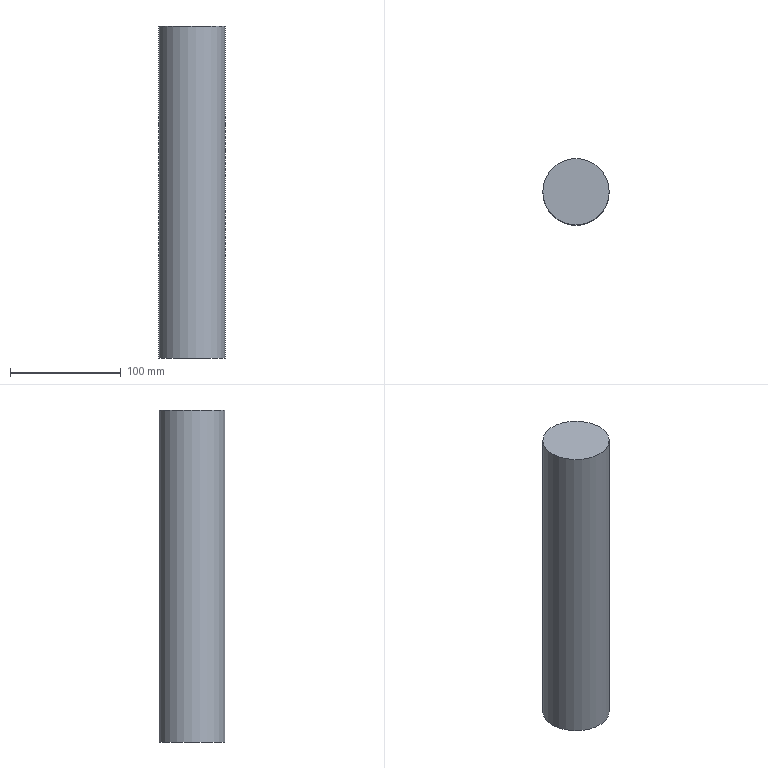Component | NX | CONNECTING_ROD | 1 solid | 3 faces | box 60 x 60 x 300 mm | volume 848230 mm3 | plane 2 | cylinder 1 | commonest cylinder face diameters 60 x1
STEP:
#1=CARTESIAN_POINT('',(0.,0.,0.));
#2=DIRECTION('',(0.,0.,1.));
#3=DIRECTION('',(1.,0.,0.));
#4=AXIS2_PLACEMENT_3D('',#1,#2,#3);
#5=CARTESIAN_POINT('',(30.,0.,-672.5));
#6=VERTEX_POINT('',#5);
#7=CARTESIAN_POINT('',(0.,0.,-672.5));
#8=DIRECTION('',(0.,0.,1.));
#9=DIRECTION('',(1.,0.,0.));
#10=AXIS2_PLACEMENT_3D('',#7,#8,#9);
#11=CIRCLE('',#10,30.);
#12=CARTESIAN_POINT('',(0.,0.,-672.5));
#13=DIRECTION('',(0.,0.,-1.));
#14=DIRECTION('',(1.,0.,0.));
#15=AXIS2_PLACEMENT_3D('',#12,#13,#14);
#16=PLANE('',#15);
#17=CARTESIAN_POINT('',(30.,0.));
#18=CARTESIAN_POINT('',(30.,-51.962));
#19=CARTESIAN_POINT('',(-15.,-25.981));
#20=CARTESIAN_POINT('',(-60.,-0.));
#21=CARTESIAN_POINT('',(-15.,25.981));
#22=CARTESIAN_POINT('',(30.,51.962));
#23=CARTESIAN_POINT('',(30.,0.));
#24=(BOUNDED_CURVE()B_SPLINE_CURVE(2,(#17,#18,#19,#20,#21,#22,#23),.UNSPECIFIED.,.T.,.F.)B_SPLINE_CURVE_WITH_KNOTS((1,2,2,2,2,1),(-2.094,0.,2.094,4.189,6.283,8.378),.UNSPECIFIED.)CURVE()GEOMETRIC_REPRESENTATION_ITEM()RATIONAL_B_SPLINE_CURVE((1.,0.5,1.,0.5,1.,0.5,1.))REPRESENTATION_ITEM(''));
#25=(GEOMETRIC_REPRESENTATION_CONTEXT(2)PARAMETRIC_REPRESENTATION_CONTEXT()REPRESENTATION_CONTEXT('',''));
#26=DEFINITIONAL_REPRESENTATION('',(#24),#25);
#27=PCURVE('',#16,#26);
#28=CARTESIAN_POINT('',(0.,0.,-372.5));
#29=DIRECTION('',(0.,0.,-1.));
#30=DIRECTION('',(1.,0.,0.));
#31=AXIS2_PLACEMENT_3D('',#28,#29,#30);
#32=CYLINDRICAL_SURFACE('',#31,30.);
#33=CARTESIAN_POINT('',(6.283,300.));
#34=DIRECTION('',(-1.,0.));
#35=VECTOR('',#34,1.);
#36=LINE('',#33,#35);
#37=(GEOMETRIC_REPRESENTATION_CONTEXT(2)PARAMETRIC_REPRESENTATION_CONTEXT()REPRESENTATION_CONTEXT('',''));
#38=DEFINITIONAL_REPRESENTATION('',(#36),#37);
#39=PCURVE('',#32,#38);
#40=SURFACE_CURVE('',#11,(#27,#39),.PCURVE_S1.);
#41=EDGE_CURVE('',#6,#6,#40,.T.);
#42=ORIENTED_EDGE('',*,*,#41,.F.);
#43=EDGE_LOOP('',(#42));
#44=FACE_BOUND('',#43,.T.);
#45=ADVANCED_FACE('',(#44),#16,.T.);
#46=CARTESIAN_POINT('',(30.,0.,-372.5));
#47=VERTEX_POINT('',#46);
#48=CARTESIAN_POINT('',(0.,0.,-372.5));
#49=DIRECTION('',(0.,0.,-1.));
#50=DIRECTION('',(1.,0.,0.));
#51=AXIS2_PLACEMENT_3D('',#48,#49,#50);
#52=CIRCLE('',#51,30.);
#53=CARTESIAN_POINT('',(0.,0.,-372.5));
#54=DIRECTION('',(0.,0.,1.));
#55=DIRECTION('',(-1.,0.,0.));
#56=AXIS2_PLACEMENT_3D('',#53,#54,#55);
#57=PLANE('',#56);
#58=CARTESIAN_POINT('',(-30.,0.));
#59=CARTESIAN_POINT('',(-30.,51.962));
#60=CARTESIAN_POINT('',(15.,25.981));
#61=CARTESIAN_POINT('',(60.,0.));
#62=CARTESIAN_POINT('',(15.,-25.981));
#63=CARTESIAN_POINT('',(-30.,-51.962));
#64=CARTESIAN_POINT('',(-30.,0.));
#65=(BOUNDED_CURVE()B_SPLINE_CURVE(2,(#58,#59,#60,#61,#62,#63,#64),.UNSPECIFIED.,.T.,.F.)B_SPLINE_CURVE_WITH_KNOTS((1,2,2,2,2,1),(-2.094,0.,2.094,4.189,6.283,8.378),.UNSPECIFIED.)CURVE()GEOMETRIC_REPRESENTATION_ITEM()RATIONAL_B_SPLINE_CURVE((1.,0.5,1.,0.5,1.,0.5,1.))REPRESENTATION_ITEM(''));
#66=(GEOMETRIC_REPRESENTATION_CONTEXT(2)PARAMETRIC_REPRESENTATION_CONTEXT()REPRESENTATION_CONTEXT('',''));
#67=DEFINITIONAL_REPRESENTATION('',(#65),#66);
#68=PCURVE('',#57,#67);
#69=CARTESIAN_POINT('',(0.,0.));
#70=DIRECTION('',(1.,0.));
#71=VECTOR('',#70,1.);
#72=LINE('',#69,#71);
#73=(GEOMETRIC_REPRESENTATION_CONTEXT(2)PARAMETRIC_REPRESENTATION_CONTEXT()REPRESENTATION_CONTEXT('',''));
#74=DEFINITIONAL_REPRESENTATION('',(#72),#73);
#75=PCURVE('',#32,#74);
#76=SURFACE_CURVE('',#52,(#68,#75),.PCURVE_S1.);
#77=EDGE_CURVE('',#47,#47,#76,.T.);
#78=ORIENTED_EDGE('',*,*,#77,.F.);
#79=EDGE_LOOP('',(#78));
#80=FACE_BOUND('',#79,.T.);
#81=ADVANCED_FACE('',(#80),#57,.T.);
#82=ORIENTED_EDGE('',*,*,#41,.T.);
#83=CARTESIAN_POINT('',(30.,0.,-372.5));
#84=CARTESIAN_POINT('',(30.,0.,-672.5));
#85=B_SPLINE_CURVE_WITH_KNOTS('',1,(#83,#84),.UNSPECIFIED.,.F.,.F.,(2,2),(0.,300.),.PIECEWISE_BEZIER_KNOTS.);
#86=CARTESIAN_POINT('',(0.,0.));
#87=DIRECTION('',(0.,1.));
#88=VECTOR('',#87,1.);
#89=LINE('',#86,#88);
#90=(GEOMETRIC_REPRESENTATION_CONTEXT(2)PARAMETRIC_REPRESENTATION_CONTEXT()REPRESENTATION_CONTEXT('',''));
#91=DEFINITIONAL_REPRESENTATION('',(#89),#90);
#92=PCURVE('',#32,#91);
#93=CARTESIAN_POINT('',(6.283,0.));
#94=DIRECTION('',(0.,1.));
#95=VECTOR('',#94,1.);
#96=LINE('',#93,#95);
#97=(GEOMETRIC_REPRESENTATION_CONTEXT(2)PARAMETRIC_REPRESENTATION_CONTEXT()REPRESENTATION_CONTEXT('',''));
#98=DEFINITIONAL_REPRESENTATION('',(#96),#97);
#99=PCURVE('',#32,#98);
#100=SEAM_CURVE('',#85,(#92,#99),.PCURVE_S1.);
#101=EDGE_CURVE('',#47,#6,#100,.T.);
#102=ORIENTED_EDGE('',*,*,#101,.F.);
#103=ORIENTED_EDGE('',*,*,#77,.T.);
#104=ORIENTED_EDGE('',*,*,#101,.T.);
#105=EDGE_LOOP('',(#82,#102,#103,#104));
#106=FACE_BOUND('',#105,.T.);
#107=ADVANCED_FACE('',(#106),#32,.T.);
#108=CLOSED_SHELL('',(#45,#81,#107));
#109=MANIFOLD_SOLID_BREP('',#108);
#110=(LENGTH_UNIT()NAMED_UNIT(*)SI_UNIT(.MILLI.,.METRE.));
#111=UNCERTAINTY_MEASURE_WITH_UNIT(LENGTH_MEASURE(0.00001),#110,'','');
#112=(NAMED_UNIT(*)PLANE_ANGLE_UNIT()SI_UNIT($,.RADIAN.));
#113=(NAMED_UNIT(*)SI_UNIT($,.STERADIAN.)SOLID_ANGLE_UNIT());
#114=(GEOMETRIC_REPRESENTATION_CONTEXT(3)GLOBAL_UNCERTAINTY_ASSIGNED_CONTEXT((#111))GLOBAL_UNIT_ASSIGNED_CONTEXT((#110,#112,#113))REPRESENTATION_CONTEXT('',''));
#115=ADVANCED_BREP_SHAPE_REPRESENTATION('',(#4,#109),#114);